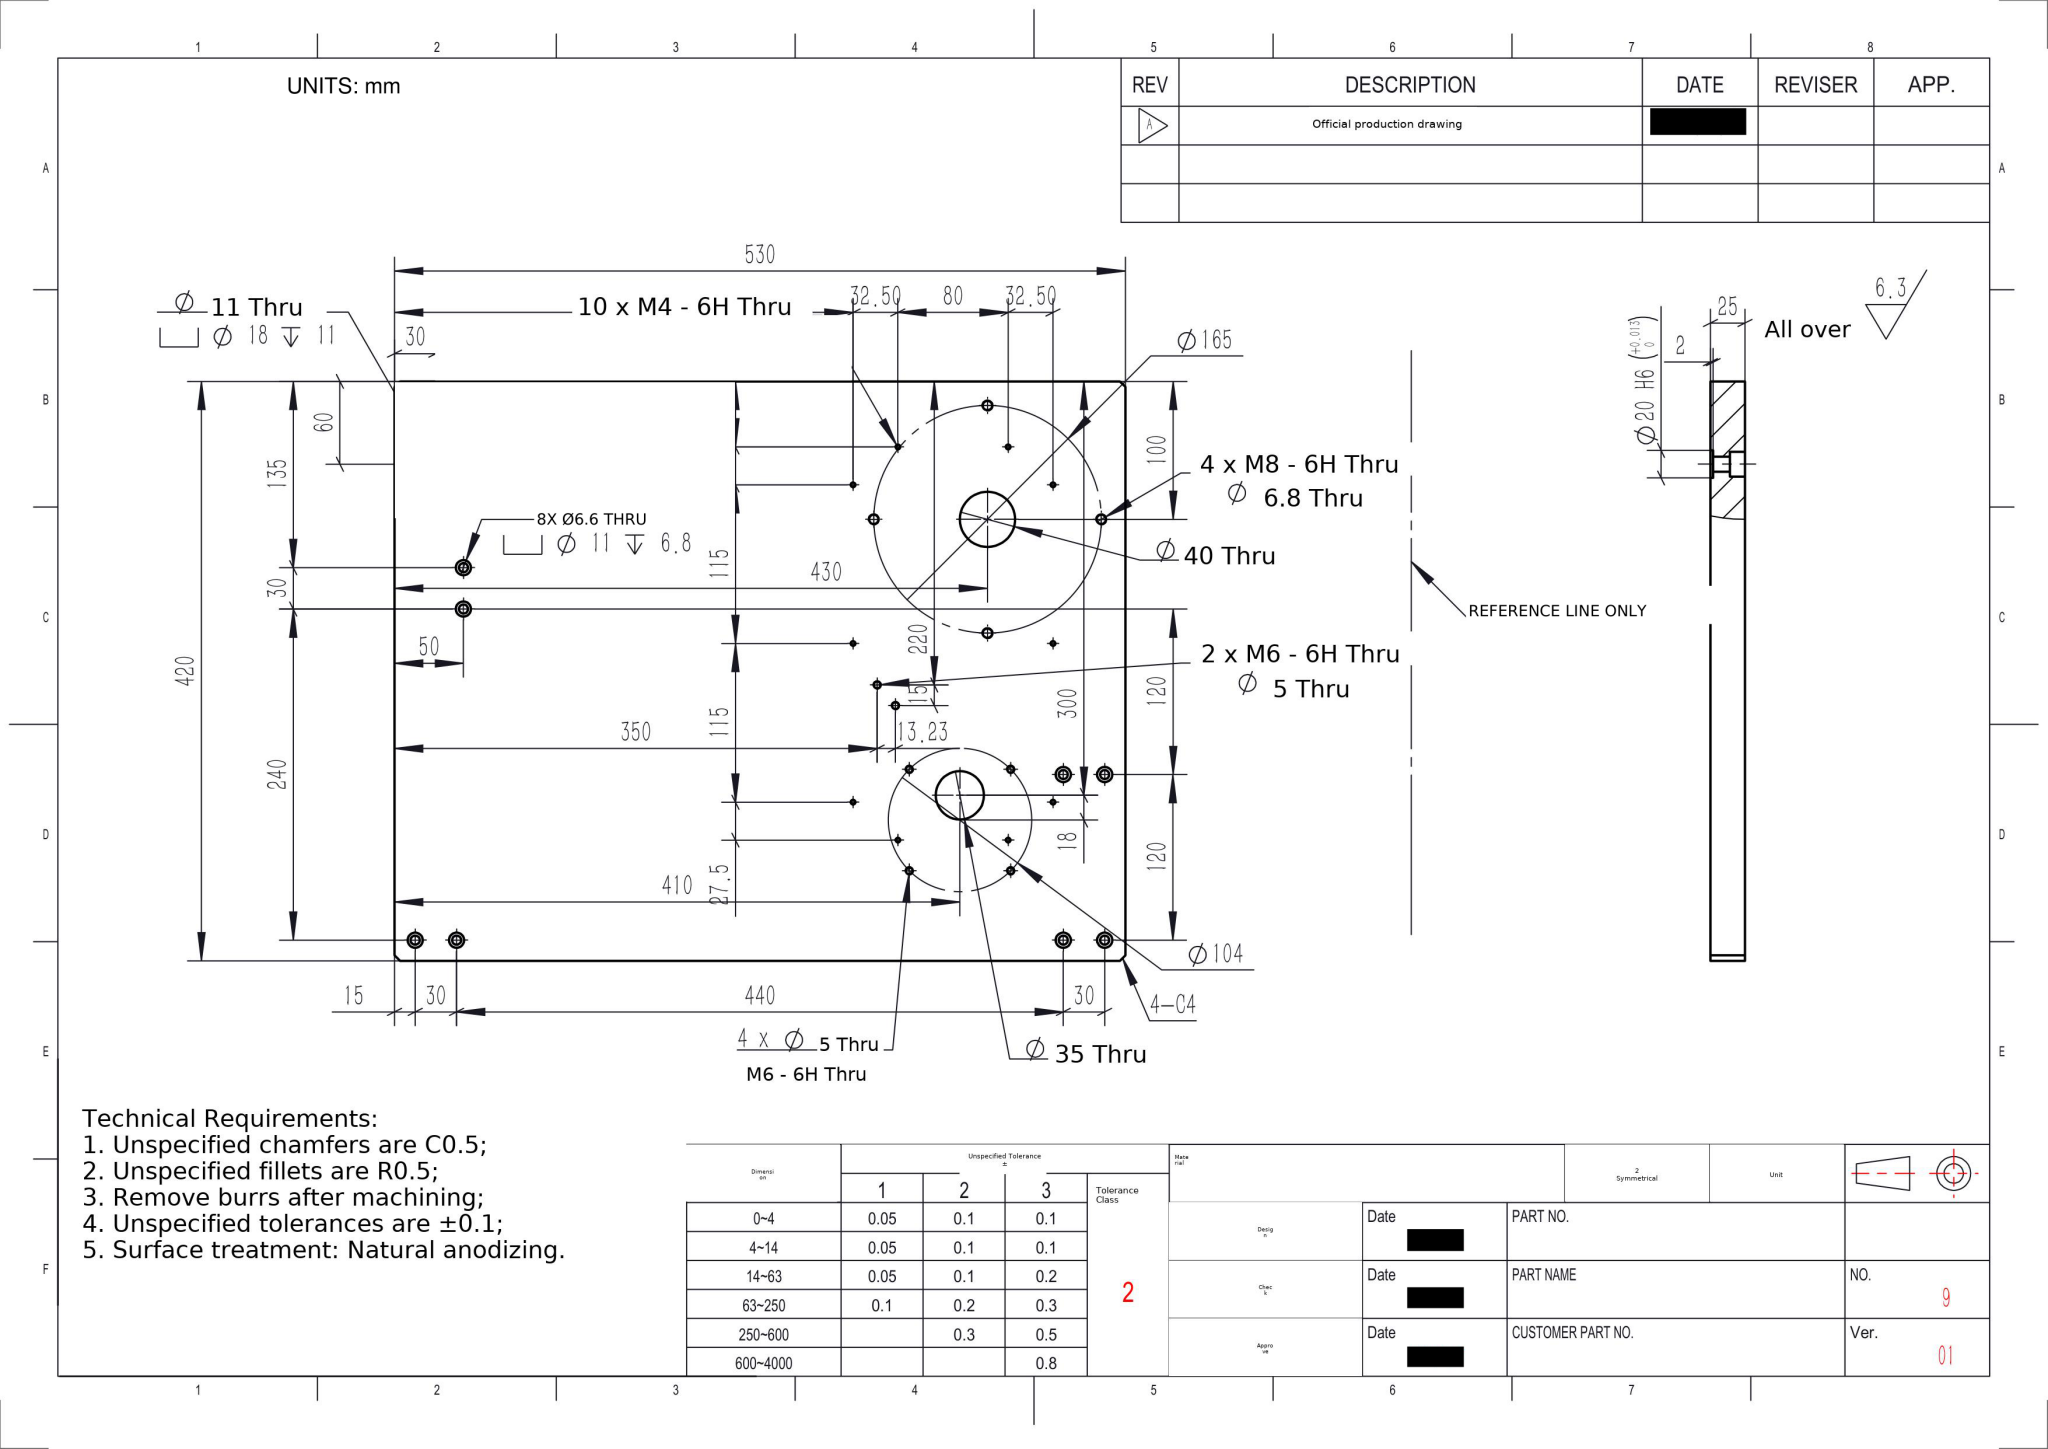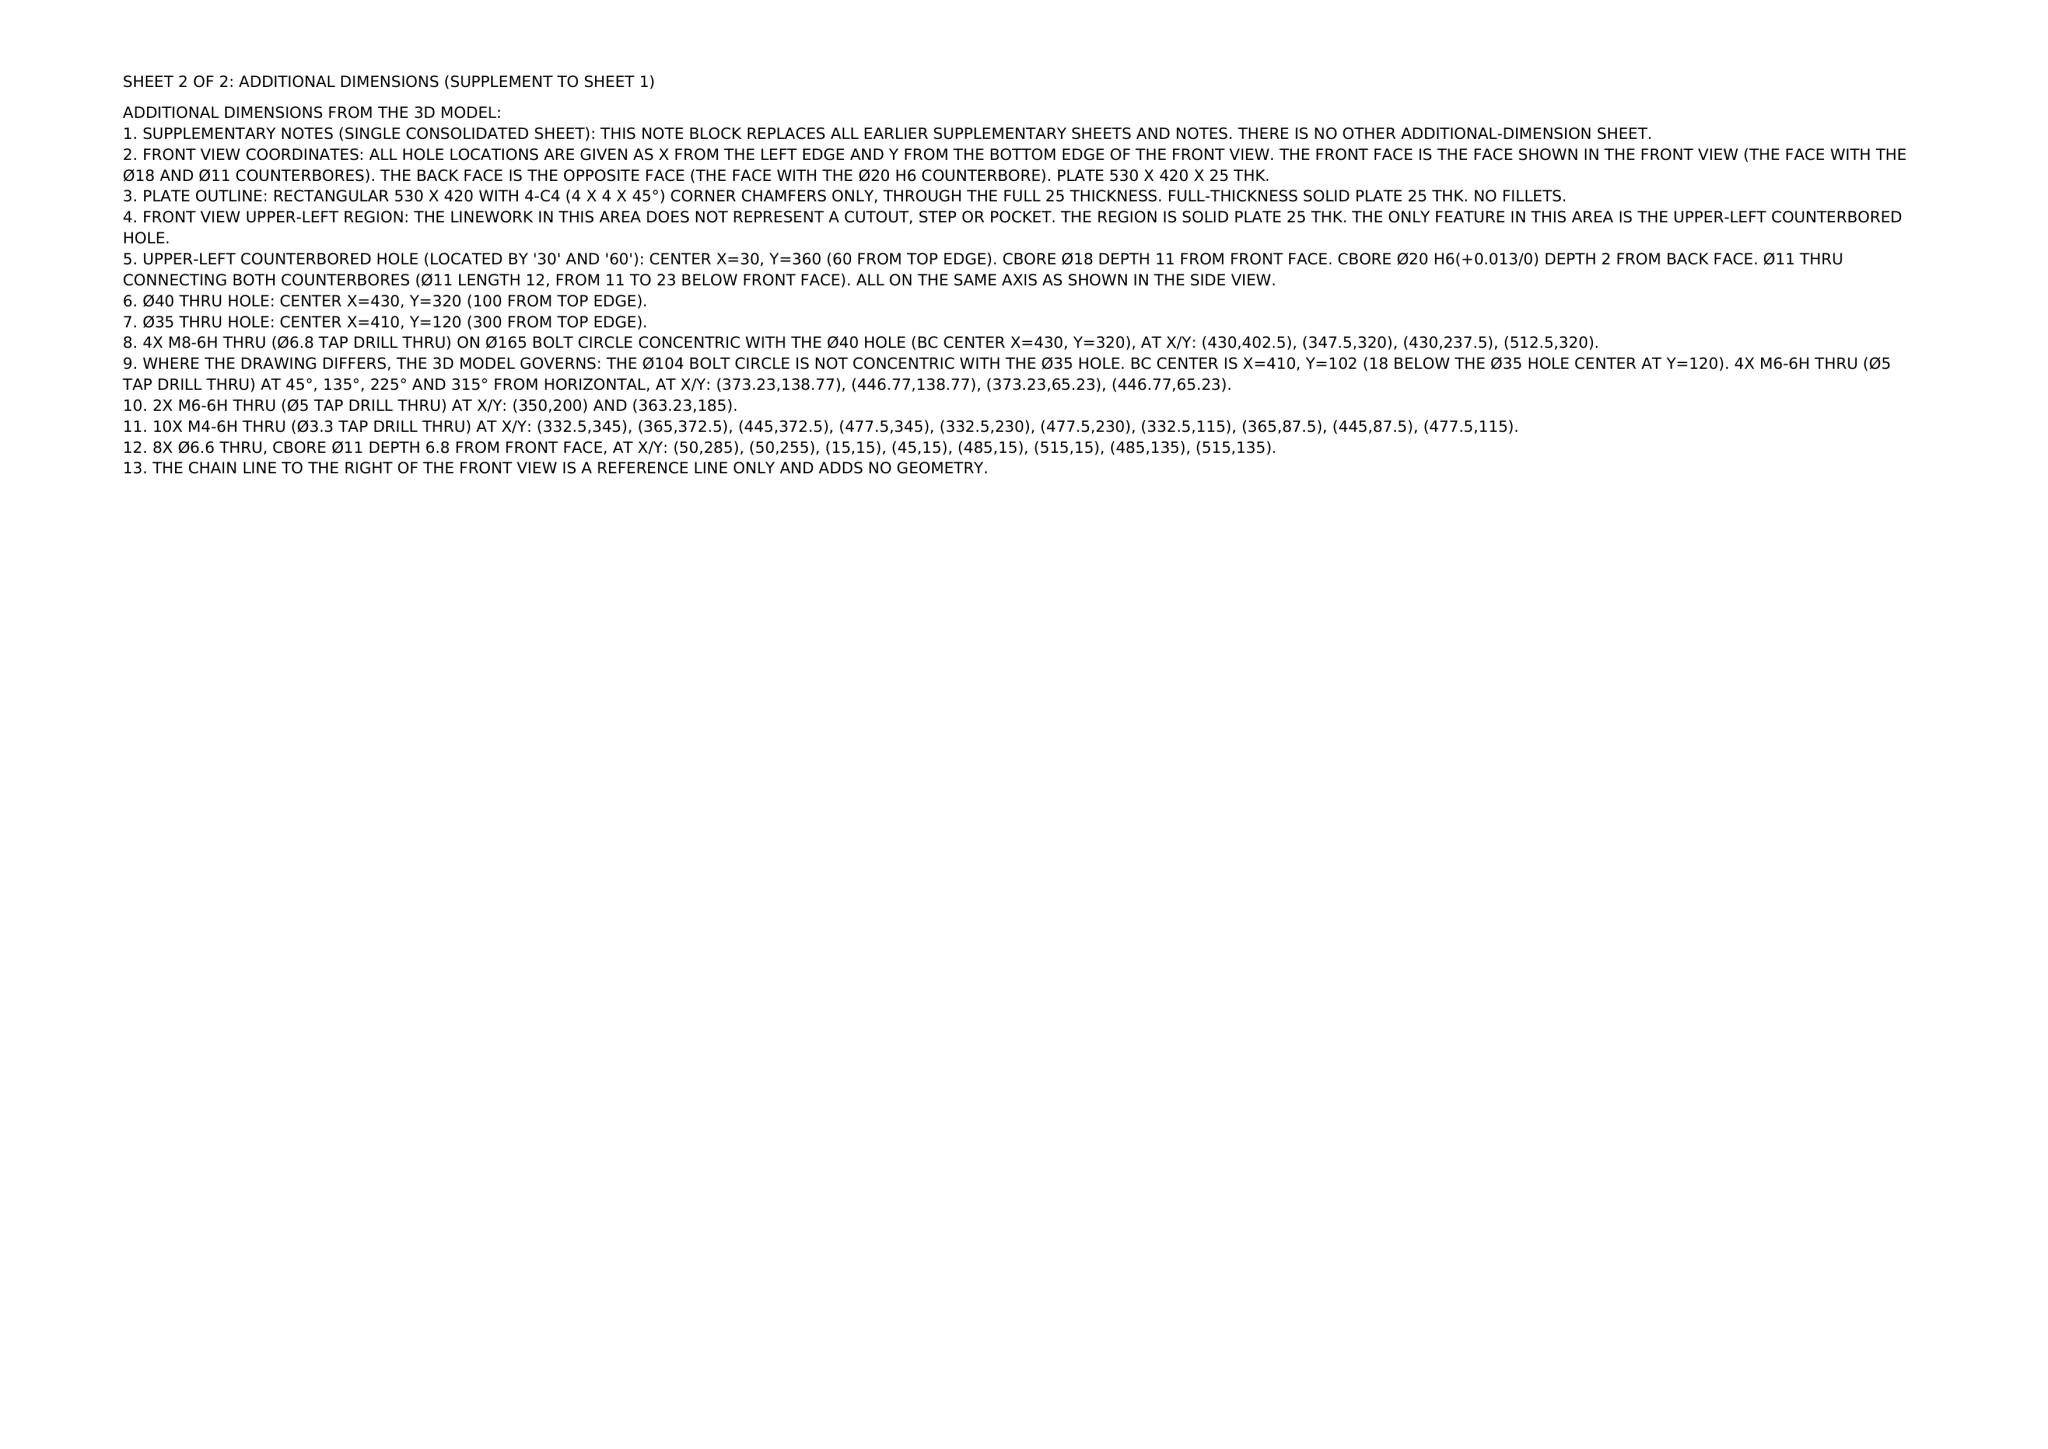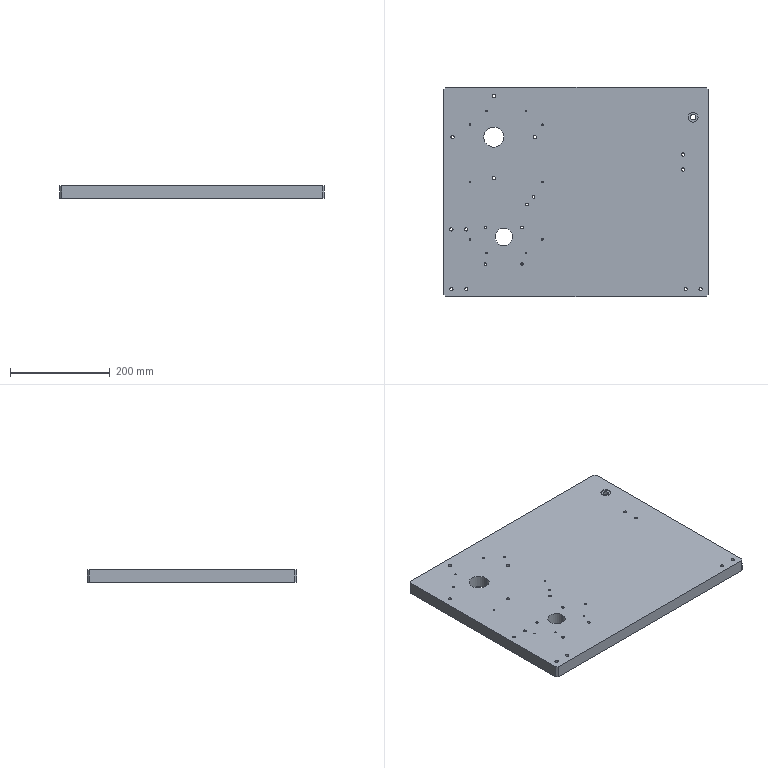Part | NX | mm | 1 solid | 102 faces | box 530 x 420 x 25 mm | volume 5485297 mm3 | cylinder 82 | plane 20 | commonest cylinder face diameters 3.3 x20 11 x18 6.6 x16 5 x12 6.8 x8 20 x2 18 x2 40 x2